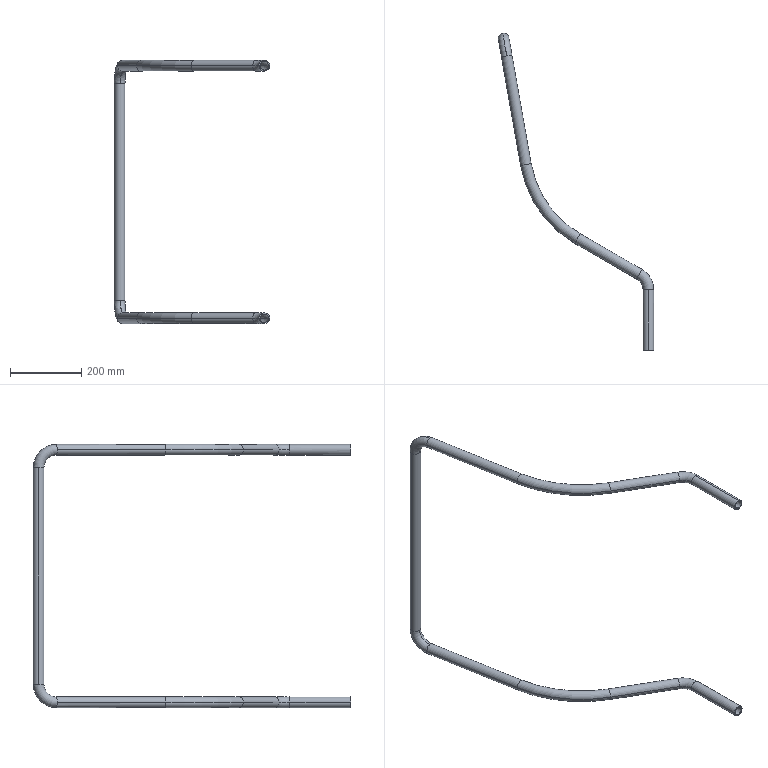Component | SolidWorks | 02-02Handrail-1 | 1 solid | 54 faces | box 436.82 x 892.16 x 740 mm | volume 702173 mm3 | cylinder 28 | torus 24 | plane 2 | commonest cylinder face diameters 24 x14 30 x14
build123d program:
from build123d import *

# Parameters (mm, degrees)
SCAN_THIN_FEATURE1_PROFILE_R   = 15
SCAN_THIN_FEATURE1_PROFILE_R_2 = 12


with BuildPart() as part:
    # Scan-Thin Feature1: sweep along a curve in space
    with BuildLine() as scan_thin_feature1_path:
        Line((0, 0, 0), (0, 171.132, 0))
        ThreePointArc((-25, 214.434, 0), (-6.699, 196.132, 0), (0, 171.132, 0))
        Line((-25, 214.434, 0), (-198.85, 314.806, 0))
        ThreePointArc((-344.292, 522.519, 0), (-294.595, 402.541, 0), (-198.85, 314.806, 0))
        Line((-344.292, 522.519, 0), (-398.142, 827.916, 0))
        ThreePointArc((-398.142, 827.916, 0), (-404.281, 862.734, -14.645), (-406.824, 877.156, -50))
        Line((-406.824, 877.156, -50), (-406.824, 877.156, -660))
        ThreePointArc((-398.142, 827.916, -710), (-404.281, 862.734, -695.355), (-406.824, 877.156, -660))
        Line((-398.142, 827.916, -710), (-344.292, 522.519, -710))
        ThreePointArc((-344.292, 522.519, -710), (-294.595, 402.541, -710), (-198.85, 314.806, -710))
        Line((-198.85, 314.806, -710), (-25, 214.434, -710))
        ThreePointArc((0, 171.132, -710), (-6.699, 196.132, -710), (-25, 214.434, -710))
        Line((0, 171.132, -710), (0, 0, -710))
    # Scan-Thin Feature1 profile (on start of the path) → Scan-Thin Feature1 (sweep)
    with BuildSketch(Plane.ZX):
        Circle(SCAN_THIN_FEATURE1_PROFILE_R)
        Circle(SCAN_THIN_FEATURE1_PROFILE_R_2, mode=Mode.SUBTRACT)
    sweep(path=scan_thin_feature1_path.line)


solid = part.part

# Placed as in the assembly
solid = solid.moved(Location((-295, 43, 355), (0, 0, 0)))